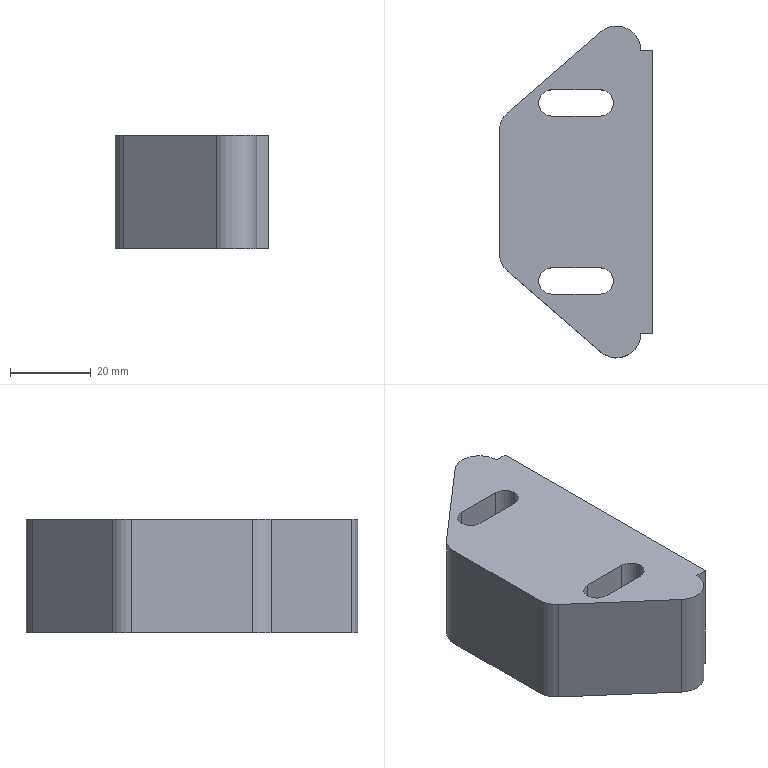Component | SolidWorks | SynchronousBeltPressingBlock-1 | 1 solid | 21 faces | box 37.99 x 82 x 28 mm | volume 62042 mm3 | plane 12 | cylinder 9 | commonest cylinder face diameters 12 x5 6.5 x4
build123d program:
from build123d import *

# Parameters (mm, degrees)
BOSS_EXTRUDE1_DEPTH              = 28
SKETCH1_W                        = 70
SKETCH1_H                        = 3.49
PRESSING_SURFACE_EXTENSION_DEPTH = 14


with BuildPart() as part:
    # Sketch1_2 → Boss-Extrude1 (new body)
    with BuildSketch(Plane(origin=(0, 0, -14), x_dir=(-1, 0, 0), z_dir=(0, 0, -1))):
        with BuildLine():
            Line((35, 0), (-35, 0))
            ThreePointArc((-35, 0), (-40.46, -3.512), (-39.528, -9.937))
            Line((-39.528, -9.937), (-19.528, -32.937))
            ThreePointArc((-19.528, -32.937), (-17.488, -34.46), (-15, -35))
            Line((-15, -35), (15, -35))
            ThreePointArc((15, -35), (17.488, -34.46), (19.528, -32.937))
            Line((19.528, -32.937), (39.528, -9.937))
            ThreePointArc((39.528, -9.937), (40.46, -3.512), (35, 0))
        make_face()
        with BuildLine():
            Line((18.75, -22), (18.75, -10))
            ThreePointArc((18.75, -10), (22, -6.75), (25.25, -10))
            Line((25.25, -10), (25.25, -22))
            ThreePointArc((25.25, -22), (22, -25.25), (18.75, -22))
        make_face(mode=Mode.SUBTRACT)
        with BuildLine():
            Line((-25.25, -22), (-25.25, -10))
            ThreePointArc((-25.25, -10), (-22, -6.75), (-18.75, -10))
            Line((-18.75, -10), (-18.75, -22))
            ThreePointArc((-18.75, -22), (-22, -25.25), (-25.25, -22))
        make_face(mode=Mode.SUBTRACT)
    extrude(amount=-BOSS_EXTRUDE1_DEPTH)

    # Sketch1 → Pressing Surface Extension (add, symmetric)
    with BuildSketch(Plane.XY):
        with Locations((0, 1.245)):
            Rectangle(SKETCH1_W, SKETCH1_H)
    extrude(amount=PRESSING_SURFACE_EXTENSION_DEPTH, both=True)


solid = part.part

# Placed as in the assembly
solid = solid.moved(Location((-60.431, 269, 134), (0, 0, -90)))
STEP:
#1=COLOUR_RGB('',0.7922,0.8196,0.9333);
#2=FILL_AREA_STYLE_COLOUR('',#1);
#3=FILL_AREA_STYLE('',(#2));
#4=SURFACE_STYLE_FILL_AREA(#3);
#5=SURFACE_SIDE_STYLE('',(#4));
#6=SURFACE_STYLE_USAGE(.BOTH.,#5);
#7=PRESENTATION_STYLE_ASSIGNMENT((#6));
#8=CARTESIAN_POINT('',(-2.77,12.147,5.827));
#9=VERTEX_POINT('',#8);
#10=CARTESIAN_POINT('',(-2.615,12.205,5.827));
#11=VERTEX_POINT('',#10);
#12=CARTESIAN_POINT('',(-2.615,11.969,5.827));
#13=DIRECTION('',(0.,0.,-1.));
#14=DIRECTION('',(0.,1.,0.));
#15=AXIS2_PLACEMENT_3D('',#12,#13,#14);
#16=CIRCLE('',#15,0.2362);
#17=EDGE_CURVE('',#9,#11,#16,.T.);
#18=ORIENTED_EDGE('',*,*,#17,.T.);
#19=CARTESIAN_POINT('',(-2.615,12.205,4.724));
#20=VERTEX_POINT('',#19);
#21=CARTESIAN_POINT('',(-2.615,12.205,5.827));
#22=DIRECTION('',(0.,0.,-1.));
#23=VECTOR('',#22,39.37);
#24=LINE('',#21,#23);
#25=EDGE_CURVE('',#11,#20,#24,.T.);
#26=ORIENTED_EDGE('',*,*,#25,.T.);
#27=CARTESIAN_POINT('',(-2.77,12.147,4.724));
#28=VERTEX_POINT('',#27);
#29=CARTESIAN_POINT('',(-2.615,11.969,4.724));
#30=DIRECTION('',(0.,0.,-1.));
#31=DIRECTION('',(0.,1.,0.));
#32=AXIS2_PLACEMENT_3D('',#29,#30,#31);
#33=CIRCLE('',#32,0.2362);
#34=EDGE_CURVE('',#28,#20,#33,.T.);
#35=ORIENTED_EDGE('',*,*,#34,.F.);
#36=CARTESIAN_POINT('',(-2.77,12.147,5.827));
#37=DIRECTION('',(0.,0.,-1.));
#38=VECTOR('',#37,39.37);
#39=LINE('',#36,#38);
#40=EDGE_CURVE('',#9,#28,#39,.T.);
#41=ORIENTED_EDGE('',*,*,#40,.F.);
#42=EDGE_LOOP('',(#18,#26,#35,#41));
#43=FACE_OUTER_BOUND('',#42,.T.);
#44=CARTESIAN_POINT('',(-2.615,11.969,5.827));
#45=DIRECTION('',(0.,0.,-1.));
#46=DIRECTION('',(0.,1.,0.));
#47=AXIS2_PLACEMENT_3D('',#44,#45,#46);
#48=CYLINDRICAL_SURFACE('',#47,0.2362);
#49=ADVANCED_FACE('',(#43),#48,.T.);
#50=ORIENTED_EDGE('',*,*,#25,.F.);
#51=CARTESIAN_POINT('',(-2.379,11.969,5.827));
#52=VERTEX_POINT('',#51);
#53=CARTESIAN_POINT('',(-2.615,11.969,5.827));
#54=DIRECTION('',(0.,0.,-1.));
#55=DIRECTION('',(0.,1.,0.));
#56=AXIS2_PLACEMENT_3D('',#53,#54,#55);
#57=CIRCLE('',#56,0.2362);
#58=EDGE_CURVE('',#11,#52,#57,.T.);
#59=ORIENTED_EDGE('',*,*,#58,.T.);
#60=CARTESIAN_POINT('',(-2.379,11.969,4.724));
#61=VERTEX_POINT('',#60);
#62=CARTESIAN_POINT('',(-2.379,11.969,5.827));
#63=DIRECTION('',(0.,0.,-1.));
#64=VECTOR('',#63,39.37);
#65=LINE('',#62,#64);
#66=EDGE_CURVE('',#52,#61,#65,.T.);
#67=ORIENTED_EDGE('',*,*,#66,.T.);
#68=CARTESIAN_POINT('',(-2.615,11.969,4.724));
#69=DIRECTION('',(0.,0.,-1.));
#70=DIRECTION('',(0.,1.,0.));
#71=AXIS2_PLACEMENT_3D('',#68,#69,#70);
#72=CIRCLE('',#71,0.2362);
#73=EDGE_CURVE('',#20,#61,#72,.T.);
#74=ORIENTED_EDGE('',*,*,#73,.F.);
#75=EDGE_LOOP('',(#50,#59,#67,#74));
#76=FACE_OUTER_BOUND('',#75,.T.);
#77=CARTESIAN_POINT('',(-2.615,11.969,5.827));
#78=DIRECTION('',(0.,0.,-1.));
#79=DIRECTION('',(0.,1.,0.));
#80=AXIS2_PLACEMENT_3D('',#77,#78,#79);
#81=CYLINDRICAL_SURFACE('',#80,0.2362);
#82=ADVANCED_FACE('',(#76),#81,.T.);
#83=CARTESIAN_POINT('',(-3.676,11.359,4.724));
#84=VERTEX_POINT('',#83);
#85=CARTESIAN_POINT('',(-3.676,11.359,4.724));
#86=DIRECTION('',(0.7546,0.6562,0.));
#87=VECTOR('',#86,39.37);
#88=LINE('',#85,#87);
#89=EDGE_CURVE('',#84,#28,#88,.T.);
#90=ORIENTED_EDGE('',*,*,#89,.F.);
#91=CARTESIAN_POINT('',(-3.676,11.359,5.827));
#92=VERTEX_POINT('',#91);
#93=CARTESIAN_POINT('',(-3.676,11.359,5.827));
#94=DIRECTION('',(0.,0.,-1.));
#95=VECTOR('',#94,39.37);
#96=LINE('',#93,#95);
#97=EDGE_CURVE('',#92,#84,#96,.T.);
#98=ORIENTED_EDGE('',*,*,#97,.F.);
#99=CARTESIAN_POINT('',(-3.676,11.359,5.827));
#100=DIRECTION('',(0.7546,0.6562,0.));
#101=VECTOR('',#100,39.37);
#102=LINE('',#99,#101);
#103=EDGE_CURVE('',#92,#9,#102,.T.);
#104=ORIENTED_EDGE('',*,*,#103,.T.);
#105=ORIENTED_EDGE('',*,*,#40,.T.);
#106=EDGE_LOOP('',(#90,#98,#104,#105));
#107=FACE_OUTER_BOUND('',#106,.T.);
#108=CARTESIAN_POINT('',(-3.676,11.359,5.827));
#109=DIRECTION('',(-0.6562,0.7546,0.));
#110=DIRECTION('',(-0.7546,-0.6562,0.));
#111=AXIS2_PLACEMENT_3D('',#108,#109,#110);
#112=PLANE('',#111);
#113=ADVANCED_FACE('',(#107),#112,.T.);
#114=CARTESIAN_POINT('',(-3.757,11.181,4.724));
#115=VERTEX_POINT('',#114);
#116=CARTESIAN_POINT('',(-3.521,11.181,4.724));
#117=DIRECTION('',(0.,0.,-1.));
#118=DIRECTION('',(0.,1.,0.));
#119=AXIS2_PLACEMENT_3D('',#116,#117,#118);
#120=CIRCLE('',#119,0.2362);
#121=EDGE_CURVE('',#115,#84,#120,.T.);
#122=ORIENTED_EDGE('',*,*,#121,.F.);
#123=CARTESIAN_POINT('',(-3.757,11.181,5.827));
#124=VERTEX_POINT('',#123);
#125=CARTESIAN_POINT('',(-3.757,11.181,5.827));
#126=DIRECTION('',(0.,0.,-1.));
#127=VECTOR('',#126,39.37);
#128=LINE('',#125,#127);
#129=EDGE_CURVE('',#124,#115,#128,.T.);
#130=ORIENTED_EDGE('',*,*,#129,.F.);
#131=CARTESIAN_POINT('',(-3.521,11.181,5.827));
#132=DIRECTION('',(0.,0.,-1.));
#133=DIRECTION('',(0.,1.,0.));
#134=AXIS2_PLACEMENT_3D('',#131,#132,#133);
#135=CIRCLE('',#134,0.2362);
#136=EDGE_CURVE('',#124,#92,#135,.T.);
#137=ORIENTED_EDGE('',*,*,#136,.T.);
#138=ORIENTED_EDGE('',*,*,#97,.T.);
#139=EDGE_LOOP('',(#122,#130,#137,#138));
#140=FACE_OUTER_BOUND('',#139,.T.);
#141=CARTESIAN_POINT('',(-3.521,11.181,5.827));
#142=DIRECTION('',(0.,0.,-1.));
#143=DIRECTION('',(0.,1.,0.));
#144=AXIS2_PLACEMENT_3D('',#141,#142,#143);
#145=CYLINDRICAL_SURFACE('',#144,0.2362);
#146=ADVANCED_FACE('',(#140),#145,.T.);
#147=CARTESIAN_POINT('',(-3.757,10.,4.724));
#148=VERTEX_POINT('',#147);
#149=CARTESIAN_POINT('',(-3.757,10.,4.724));
#150=DIRECTION('',(0.,1.,0.));
#151=VECTOR('',#150,39.37);
#152=LINE('',#149,#151);
#153=EDGE_CURVE('',#148,#115,#152,.T.);
#154=ORIENTED_EDGE('',*,*,#153,.F.);
#155=CARTESIAN_POINT('',(-3.757,10.,5.827));
#156=VERTEX_POINT('',#155);
#157=CARTESIAN_POINT('',(-3.757,10.,5.827));
#158=DIRECTION('',(0.,0.,-1.));
#159=VECTOR('',#158,39.37);
#160=LINE('',#157,#159);
#161=EDGE_CURVE('',#156,#148,#160,.T.);
#162=ORIENTED_EDGE('',*,*,#161,.F.);
#163=CARTESIAN_POINT('',(-3.757,10.,5.827));
#164=DIRECTION('',(0.,1.,0.));
#165=VECTOR('',#164,39.37);
#166=LINE('',#163,#165);
#167=EDGE_CURVE('',#156,#124,#166,.T.);
#168=ORIENTED_EDGE('',*,*,#167,.T.);
#169=ORIENTED_EDGE('',*,*,#129,.T.);
#170=EDGE_LOOP('',(#154,#162,#168,#169));
#171=FACE_OUTER_BOUND('',#170,.T.);
#172=CARTESIAN_POINT('',(-3.757,10.,5.827));
#173=DIRECTION('',(-1.,0.,0.));
#174=DIRECTION('',(0.,0.,-1.));
#175=AXIS2_PLACEMENT_3D('',#172,#173,#174);
#176=PLANE('',#175);
#177=ADVANCED_FACE('',(#171),#176,.T.);
#178=CARTESIAN_POINT('',(-3.676,9.822,4.724));
#179=VERTEX_POINT('',#178);
#180=CARTESIAN_POINT('',(-3.521,10.,4.724));
#181=DIRECTION('',(0.,0.,-1.));
#182=DIRECTION('',(0.,1.,0.));
#183=AXIS2_PLACEMENT_3D('',#180,#181,#182);
#184=CIRCLE('',#183,0.2362);
#185=EDGE_CURVE('',#179,#148,#184,.T.);
#186=ORIENTED_EDGE('',*,*,#185,.F.);
#187=CARTESIAN_POINT('',(-3.676,9.822,5.827));
#188=VERTEX_POINT('',#187);
#189=CARTESIAN_POINT('',(-3.676,9.822,5.827));
#190=DIRECTION('',(0.,0.,-1.));
#191=VECTOR('',#190,39.37);
#192=LINE('',#189,#191);
#193=EDGE_CURVE('',#188,#179,#192,.T.);
#194=ORIENTED_EDGE('',*,*,#193,.F.);
#195=CARTESIAN_POINT('',(-3.521,10.,5.827));
#196=DIRECTION('',(0.,0.,-1.));
#197=DIRECTION('',(0.,1.,0.));
#198=AXIS2_PLACEMENT_3D('',#195,#196,#197);
#199=CIRCLE('',#198,0.2362);
#200=EDGE_CURVE('',#188,#156,#199,.T.);
#201=ORIENTED_EDGE('',*,*,#200,.T.);
#202=ORIENTED_EDGE('',*,*,#161,.T.);
#203=EDGE_LOOP('',(#186,#194,#201,#202));
#204=FACE_OUTER_BOUND('',#203,.T.);
#205=CARTESIAN_POINT('',(-3.521,10.,5.827));
#206=DIRECTION('',(0.,0.,-1.));
#207=DIRECTION('',(0.,1.,0.));
#208=AXIS2_PLACEMENT_3D('',#205,#206,#207);
#209=CYLINDRICAL_SURFACE('',#208,0.2362);
#210=ADVANCED_FACE('',(#204),#209,.T.);
#211=CARTESIAN_POINT('',(-2.77,9.034,4.724));
#212=VERTEX_POINT('',#211);
#213=CARTESIAN_POINT('',(-2.77,9.034,4.724));
#214=DIRECTION('',(-0.7546,0.6562,0.));
#215=VECTOR('',#214,39.37);
#216=LINE('',#213,#215);
#217=EDGE_CURVE('',#212,#179,#216,.T.);
#218=ORIENTED_EDGE('',*,*,#217,.F.);
#219=CARTESIAN_POINT('',(-2.77,9.034,5.827));
#220=VERTEX_POINT('',#219);
#221=CARTESIAN_POINT('',(-2.77,9.034,5.827));
#222=DIRECTION('',(0.,0.,-1.));
#223=VECTOR('',#222,39.37);
#224=LINE('',#221,#223);
#225=EDGE_CURVE('',#220,#212,#224,.T.);
#226=ORIENTED_EDGE('',*,*,#225,.F.);
#227=CARTESIAN_POINT('',(-2.77,9.034,5.827));
#228=DIRECTION('',(-0.7546,0.6562,0.));
#229=VECTOR('',#228,39.37);
#230=LINE('',#227,#229);
#231=EDGE_CURVE('',#220,#188,#230,.T.);
#232=ORIENTED_EDGE('',*,*,#231,.T.);
#233=ORIENTED_EDGE('',*,*,#193,.T.);
#234=EDGE_LOOP('',(#218,#226,#232,#233));
#235=FACE_OUTER_BOUND('',#234,.T.);
#236=CARTESIAN_POINT('',(-2.77,9.034,5.827));
#237=DIRECTION('',(-0.6562,-0.7546,0.));
#238=DIRECTION('',(0.7546,-0.6562,0.));
#239=AXIS2_PLACEMENT_3D('',#236,#237,#238);
#240=PLANE('',#239);
#241=ADVANCED_FACE('',(#235),#240,.T.);
#242=CARTESIAN_POINT('',(-2.379,9.213,4.724));
#243=VERTEX_POINT('',#242);
#244=CARTESIAN_POINT('',(-2.615,9.213,4.724));
#245=DIRECTION('',(0.,0.,-1.));
#246=DIRECTION('',(0.,1.,0.));
#247=AXIS2_PLACEMENT_3D('',#244,#245,#246);
#248=CIRCLE('',#247,0.2362);
#249=EDGE_CURVE('',#243,#212,#248,.T.);
#250=ORIENTED_EDGE('',*,*,#249,.F.);
#251=CARTESIAN_POINT('',(-2.379,9.213,5.827));
#252=VERTEX_POINT('',#251);
#253=CARTESIAN_POINT('',(-2.379,9.213,5.827));
#254=DIRECTION('',(0.,0.,-1.));
#255=VECTOR('',#254,39.37);
#256=LINE('',#253,#255);
#257=EDGE_CURVE('',#252,#243,#256,.T.);
#258=ORIENTED_EDGE('',*,*,#257,.F.);
#259=CARTESIAN_POINT('',(-2.615,9.213,5.827));
#260=DIRECTION('',(0.,0.,-1.));
#261=DIRECTION('',(0.,1.,0.));
#262=AXIS2_PLACEMENT_3D('',#259,#260,#261);
#263=CIRCLE('',#262,0.2362);
#264=EDGE_CURVE('',#252,#220,#263,.T.);
#265=ORIENTED_EDGE('',*,*,#264,.T.);
#266=ORIENTED_EDGE('',*,*,#225,.T.);
#267=EDGE_LOOP('',(#250,#258,#265,#266));
#268=FACE_OUTER_BOUND('',#267,.T.);
#269=CARTESIAN_POINT('',(-2.615,9.213,5.827));
#270=DIRECTION('',(0.,0.,-1.));
#271=DIRECTION('',(0.,1.,0.));
#272=AXIS2_PLACEMENT_3D('',#269,#270,#271);
#273=CYLINDRICAL_SURFACE('',#272,0.2362);
#274=ADVANCED_FACE('',(#268),#273,.T.);
#275=ORIENTED_EDGE('',*,*,#264,.F.);
#276=CARTESIAN_POINT('',(-2.261,9.213,5.827));
#277=VERTEX_POINT('',#276);
#278=CARTESIAN_POINT('',(-2.399,9.213,5.827));
#279=DIRECTION('',(1.,-0.,0.));
#280=VECTOR('',#279,39.37);
#281=LINE('',#278,#280);
#282=EDGE_CURVE('',#252,#277,#281,.T.);
#283=ORIENTED_EDGE('',*,*,#282,.T.);
#284=CARTESIAN_POINT('',(-2.261,11.969,5.827));
#285=VERTEX_POINT('',#284);
#286=CARTESIAN_POINT('',(-2.261,9.213,5.827));
#287=DIRECTION('',(0.,1.,0.));
#288=VECTOR('',#287,39.37);
#289=LINE('',#286,#288);
#290=EDGE_CURVE('',#277,#285,#289,.T.);
#291=ORIENTED_EDGE('',*,*,#290,.T.);
#292=CARTESIAN_POINT('',(-2.261,11.969,5.827));
#293=DIRECTION('',(-1.,0.,0.));
#294=VECTOR('',#293,39.37);
#295=LINE('',#292,#294);
#296=EDGE_CURVE('',#285,#52,#295,.T.);
#297=ORIENTED_EDGE('',*,*,#296,.T.);
#298=ORIENTED_EDGE('',*,*,#58,.F.);
#299=ORIENTED_EDGE('',*,*,#17,.F.);
#300=ORIENTED_EDGE('',*,*,#103,.F.);
#301=ORIENTED_EDGE('',*,*,#136,.F.);
#302=ORIENTED_EDGE('',*,*,#167,.F.);
#303=ORIENTED_EDGE('',*,*,#200,.F.);
#304=ORIENTED_EDGE('',*,*,#231,.F.);
#305=EDGE_LOOP('',(#275,#283,#291,#297,#298,#299,#300,#301,#302,#303,#304));
#306=FACE_OUTER_BOUND('',#305,.T.);
#307=CARTESIAN_POINT('',(-2.773,11.329,5.827));
#308=VERTEX_POINT('',#307);
#309=CARTESIAN_POINT('',(-3.245,11.329,5.827));
#310=VERTEX_POINT('',#309);
#311=CARTESIAN_POINT('',(-3.245,11.329,5.827));
#312=DIRECTION('',(-1.,0.,0.));
#313=VECTOR('',#312,39.37);
#314=LINE('',#311,#313);
#315=EDGE_CURVE('',#308,#310,#314,.T.);
#316=ORIENTED_EDGE('',*,*,#315,.T.);
#317=CARTESIAN_POINT('',(-3.245,11.585,5.827));
#318=VERTEX_POINT('',#317);
#319=CARTESIAN_POINT('',(-3.245,11.457,5.827));
#320=DIRECTION('',(0.,0.,-1.));
#321=DIRECTION('',(0.,-1.,0.));
#322=AXIS2_PLACEMENT_3D('',#319,#320,#321);
#323=CIRCLE('',#322,0.128);
#324=EDGE_CURVE('',#310,#318,#323,.T.);
#325=ORIENTED_EDGE('',*,*,#324,.T.);
#326=CARTESIAN_POINT('',(-2.773,11.585,5.827));
#327=VERTEX_POINT('',#326);
#328=CARTESIAN_POINT('',(-2.773,11.585,5.827));
#329=DIRECTION('',(1.,-0.,0.));
#330=VECTOR('',#329,39.37);
#331=LINE('',#328,#330);
#332=EDGE_CURVE('',#318,#327,#331,.T.);
#333=ORIENTED_EDGE('',*,*,#332,.T.);
#334=CARTESIAN_POINT('',(-2.773,11.457,5.827));
#335=DIRECTION('',(0.,0.,-1.));
#336=DIRECTION('',(0.,-1.,0.));
#337=AXIS2_PLACEMENT_3D('',#334,#335,#336);
#338=CIRCLE('',#337,0.128);
#339=EDGE_CURVE('',#327,#308,#338,.T.);
#340=ORIENTED_EDGE('',*,*,#339,.T.);
#341=EDGE_LOOP('',(#316,#325,#333,#340));
#342=FACE_BOUND('',#341,.T.);
#343=CARTESIAN_POINT('',(-2.773,9.596,5.827));
#344=VERTEX_POINT('',#343);
#345=CARTESIAN_POINT('',(-3.245,9.596,5.827));
#346=VERTEX_POINT('',#345);
#347=CARTESIAN_POINT('',(-3.245,9.596,5.827));
#348=DIRECTION('',(-1.,0.,0.));
#349=VECTOR('',#348,39.37);
#350=LINE('',#347,#349);
#351=EDGE_CURVE('',#344,#346,#350,.T.);
#352=ORIENTED_EDGE('',*,*,#351,.T.);
#353=CARTESIAN_POINT('',(-3.245,9.852,5.827));
#354=VERTEX_POINT('',#353);
#355=CARTESIAN_POINT('',(-3.245,9.724,5.827));
#356=DIRECTION('',(0.,0.,-1.));
#357=DIRECTION('',(0.,-1.,0.));
#358=AXIS2_PLACEMENT_3D('',#355,#356,#357);
#359=CIRCLE('',#358,0.128);
#360=EDGE_CURVE('',#346,#354,#359,.T.);
#361=ORIENTED_EDGE('',*,*,#360,.T.);
#362=CARTESIAN_POINT('',(-2.773,9.852,5.827));
#363=VERTEX_POINT('',#362);
#364=CARTESIAN_POINT('',(-2.773,9.852,5.827));
#365=DIRECTION('',(1.,-0.,0.));
#366=VECTOR('',#365,39.37);
#367=LINE('',#364,#366);
#368=EDGE_CURVE('',#354,#363,#367,.T.);
#369=ORIENTED_EDGE('',*,*,#368,.T.);
#370=CARTESIAN_POINT('',(-2.773,9.724,5.827));
#371=DIRECTION('',(0.,0.,-1.));
#372=DIRECTION('',(0.,-1.,0.));
#373=AXIS2_PLACEMENT_3D('',#370,#371,#372);
#374=CIRCLE('',#373,0.128);
#375=EDGE_CURVE('',#363,#344,#374,.T.);
#376=ORIENTED_EDGE('',*,*,#375,.T.);
#377=EDGE_LOOP('',(#352,#361,#369,#376));
#378=FACE_BOUND('',#377,.T.);
#379=CARTESIAN_POINT('',(-2.615,11.969,5.827));
#380=DIRECTION('',(0.,0.,-1.));
#381=DIRECTION('',(0.,1.,0.));
#382=AXIS2_PLACEMENT_3D('',#379,#380,#381);
#383=PLANE('',#382);
#384=ADVANCED_FACE('',(#306,#342,#378),#383,.F.);
#385=ORIENTED_EDGE('',*,*,#34,.T.);
#386=ORIENTED_EDGE('',*,*,#73,.T.);
#387=CARTESIAN_POINT('',(-2.261,11.969,4.724));
#388=VERTEX_POINT('',#387);
#389=CARTESIAN_POINT('',(-2.261,11.969,4.724));
#390=DIRECTION('',(-1.,0.,0.));
#391=VECTOR('',#390,39.37);
#392=LINE('',#389,#391);
#393=EDGE_CURVE('',#388,#61,#392,.T.);
#394=ORIENTED_EDGE('',*,*,#393,.F.);
#395=CARTESIAN_POINT('',(-2.261,9.213,4.724));
#396=VERTEX_POINT('',#395);
#397=CARTESIAN_POINT('',(-2.261,9.213,4.724));
#398=DIRECTION('',(0.,1.,0.));
#399=VECTOR('',#398,39.37);
#400=LINE('',#397,#399);
#401=EDGE_CURVE('',#396,#388,#400,.T.);
#402=ORIENTED_EDGE('',*,*,#401,.F.);
#403=CARTESIAN_POINT('',(-2.399,9.213,4.724));
#404=DIRECTION('',(1.,-0.,0.));
#405=VECTOR('',#404,39.37);
#406=LINE('',#403,#405);
#407=EDGE_CURVE('',#243,#396,#406,.T.);
#408=ORIENTED_EDGE('',*,*,#407,.F.);
#409=ORIENTED_EDGE('',*,*,#249,.T.);
#410=ORIENTED_EDGE('',*,*,#217,.T.);
#411=ORIENTED_EDGE('',*,*,#185,.T.);
#412=ORIENTED_EDGE('',*,*,#153,.T.);
#413=ORIENTED_EDGE('',*,*,#121,.T.);
#414=ORIENTED_EDGE('',*,*,#89,.T.);
#415=EDGE_LOOP('',(#385,#386,#394,#402,#408,#409,#410,#411,#412,#413,#414));
#416=FACE_OUTER_BOUND('',#415,.T.);
#417=CARTESIAN_POINT('',(-3.245,9.596,4.724));
#418=VERTEX_POINT('',#417);
#419=CARTESIAN_POINT('',(-3.245,9.852,4.724));
#420=VERTEX_POINT('',#419);
#421=CARTESIAN_POINT('',(-3.245,9.724,4.724));
#422=DIRECTION('',(0.,0.,-1.));
#423=DIRECTION('',(0.,-1.,0.));
#424=AXIS2_PLACEMENT_3D('',#421,#422,#423);
#425=CIRCLE('',#424,0.128);
#426=EDGE_CURVE('',#418,#420,#425,.T.);
#427=ORIENTED_EDGE('',*,*,#426,.F.);
#428=CARTESIAN_POINT('',(-2.773,9.596,4.724));
#429=VERTEX_POINT('',#428);
#430=CARTESIAN_POINT('',(-3.245,9.596,4.724));
#431=DIRECTION('',(-1.,0.,0.));
#432=VECTOR('',#431,39.37);
#433=LINE('',#430,#432);
#434=EDGE_CURVE('',#429,#418,#433,.T.);
#435=ORIENTED_EDGE('',*,*,#434,.F.);
#436=CARTESIAN_POINT('',(-2.773,9.852,4.724));
#437=VERTEX_POINT('',#436);
#438=CARTESIAN_POINT('',(-2.773,9.724,4.724));
#439=DIRECTION('',(0.,0.,-1.));
#440=DIRECTION('',(0.,-1.,0.));
#441=AXIS2_PLACEMENT_3D('',#438,#439,#440);
#442=CIRCLE('',#441,0.128);
#443=EDGE_CURVE('',#437,#429,#442,.T.);
#444=ORIENTED_EDGE('',*,*,#443,.F.);
#445=CARTESIAN_POINT('',(-2.773,9.852,4.724));
#446=DIRECTION('',(1.,-0.,0.));
#447=VECTOR('',#446,39.37);
#448=LINE('',#445,#447);
#449=EDGE_CURVE('',#420,#437,#448,.T.);
#450=ORIENTED_EDGE('',*,*,#449,.F.);
#451=EDGE_LOOP('',(#427,#435,#444,#450));
#452=FACE_BOUND('',#451,.T.);
#453=CARTESIAN_POINT('',(-3.245,11.329,4.724));
#454=VERTEX_POINT('',#453);
#455=CARTESIAN_POINT('',(-3.245,11.585,4.724));
#456=VERTEX_POINT('',#455);
#457=CARTESIAN_POINT('',(-3.245,11.457,4.724));
#458=DIRECTION('',(0.,0.,-1.));
#459=DIRECTION('',(0.,-1.,0.));
#460=AXIS2_PLACEMENT_3D('',#457,#458,#459);
#461=CIRCLE('',#460,0.128);
#462=EDGE_CURVE('',#454,#456,#461,.T.);
#463=ORIENTED_EDGE('',*,*,#462,.F.);
#464=CARTESIAN_POINT('',(-2.773,11.329,4.724));
#465=VERTEX_POINT('',#464);
#466=CARTESIAN_POINT('',(-3.245,11.329,4.724));
#467=DIRECTION('',(-1.,0.,0.));
#468=VECTOR('',#467,39.37);
#469=LINE('',#466,#468);
#470=EDGE_CURVE('',#465,#454,#469,.T.);
#471=ORIENTED_EDGE('',*,*,#470,.F.);
#472=CARTESIAN_POINT('',(-2.773,11.585,4.724));
#473=VERTEX_POINT('',#472);
#474=CARTESIAN_POINT('',(-2.773,11.457,4.724));
#475=DIRECTION('',(0.,0.,-1.));
#476=DIRECTION('',(0.,-1.,0.));
#477=AXIS2_PLACEMENT_3D('',#474,#475,#476);
#478=CIRCLE('',#477,0.128);
#479=EDGE_CURVE('',#473,#465,#478,.T.);
#480=ORIENTED_EDGE('',*,*,#479,.F.);
#481=CARTESIAN_POINT('',(-2.773,11.585,4.724));
#482=DIRECTION('',(1.,-0.,0.));
#483=VECTOR('',#482,39.37);
#484=LINE('',#481,#483);
#485=EDGE_CURVE('',#456,#473,#484,.T.);
#486=ORIENTED_EDGE('',*,*,#485,.F.);
#487=EDGE_LOOP('',(#463,#471,#480,#486));
#488=FACE_BOUND('',#487,.T.);
#489=CARTESIAN_POINT('',(-2.615,11.969,4.724));
#490=DIRECTION('',(0.,0.,-1.));
#491=DIRECTION('',(0.,1.,0.));
#492=AXIS2_PLACEMENT_3D('',#489,#490,#491);
#493=PLANE('',#492);
#494=ADVANCED_FACE('',(#416,#452,#488),#493,.T.);
#495=ORIENTED_EDGE('',*,*,#462,.T.);
#496=CARTESIAN_POINT('',(-3.245,11.585,5.827));
#497=DIRECTION('',(0.,0.,-1.));
#498=VECTOR('',#497,39.37);
#499=LINE('',#496,#498);
#500=EDGE_CURVE('',#318,#456,#499,.T.);
#501=ORIENTED_EDGE('',*,*,#500,.F.);
#502=ORIENTED_EDGE('',*,*,#324,.F.);
#503=CARTESIAN_POINT('',(-3.245,11.329,5.827));
#504=DIRECTION('',(0.,0.,-1.));
#505=VECTOR('',#504,39.37);
#506=LINE('',#503,#505);
#507=EDGE_CURVE('',#310,#454,#506,.T.);
#508=ORIENTED_EDGE('',*,*,#507,.T.);
#509=EDGE_LOOP('',(#495,#501,#502,#508));
#510=FACE_OUTER_BOUND('',#509,.T.);
#511=CARTESIAN_POINT('',(-3.245,11.457,5.827));
#512=DIRECTION('',(0.,0.,-1.));
#513=DIRECTION('',(0.,1.,0.));
#514=AXIS2_PLACEMENT_3D('',#511,#512,#513);
#515=CYLINDRICAL_SURFACE('',#514,0.128);
#516=ADVANCED_FACE('',(#510),#515,.F.);
#517=ORIENTED_EDGE('',*,*,#470,.T.);
#518=ORIENTED_EDGE('',*,*,#507,.F.);
#519=ORIENTED_EDGE('',*,*,#315,.F.);
#520=CARTESIAN_POINT('',(-2.773,11.329,5.827));
#521=DIRECTION('',(0.,0.,-1.));
#522=VECTOR('',#521,39.37);
#523=LINE('',#520,#522);
#524=EDGE_CURVE('',#308,#465,#523,.T.);
#525=ORIENTED_EDGE('',*,*,#524,.T.);
#526=EDGE_LOOP('',(#517,#518,#519,#525));
#527=FACE_OUTER_BOUND('',#526,.T.);
#528=CARTESIAN_POINT('',(-3.245,11.329,5.827));
#529=DIRECTION('',(-0.,-1.,0.));
#530=DIRECTION('',(0.,0.,-1.));
#531=AXIS2_PLACEMENT_3D('',#528,#529,#530);
#532=PLANE('',#531);
#533=ADVANCED_FACE('',(#527),#532,.F.);
#534=ORIENTED_EDGE('',*,*,#479,.T.);
#535=ORIENTED_EDGE('',*,*,#524,.F.);
#536=ORIENTED_EDGE('',*,*,#339,.F.);
#537=CARTESIAN_POINT('',(-2.773,11.585,5.827));
#538=DIRECTION('',(0.,0.,-1.));
#539=VECTOR('',#538,39.37);
#540=LINE('',#537,#539);
#541=EDGE_CURVE('',#327,#473,#540,.T.);
#542=ORIENTED_EDGE('',*,*,#541,.T.);
#543=EDGE_LOOP('',(#534,#535,#536,#542));
#544=FACE_OUTER_BOUND('',#543,.T.);
#545=CARTESIAN_POINT('',(-2.773,11.457,5.827));
#546=DIRECTION('',(0.,0.,-1.));
#547=DIRECTION('',(0.,1.,0.));
#548=AXIS2_PLACEMENT_3D('',#545,#546,#547);
#549=CYLINDRICAL_SURFACE('',#548,0.128);
#550=ADVANCED_FACE('',(#544),#549,.F.);
#551=ORIENTED_EDGE('',*,*,#485,.T.);
#552=ORIENTED_EDGE('',*,*,#541,.F.);
#553=ORIENTED_EDGE('',*,*,#332,.F.);
#554=ORIENTED_EDGE('',*,*,#500,.T.);
#555=EDGE_LOOP('',(#551,#552,#553,#554));
#556=FACE_OUTER_BOUND('',#555,.T.);
#557=CARTESIAN_POINT('',(-2.773,11.585,5.827));
#558=DIRECTION('',(0.,1.,0.));
#559=DIRECTION('',(0.,0.,1.));
#560=AXIS2_PLACEMENT_3D('',#557,#558,#559);
#561=PLANE('',#560);
#562=ADVANCED_FACE('',(#556),#561,.F.);
#563=ORIENTED_EDGE('',*,*,#426,.T.);
#564=CARTESIAN_POINT('',(-3.245,9.852,5.827));
#565=DIRECTION('',(0.,0.,-1.));
#566=VECTOR('',#565,39.37);
#567=LINE('',#564,#566);
#568=EDGE_CURVE('',#354,#420,#567,.T.);
#569=ORIENTED_EDGE('',*,*,#568,.F.);
#570=ORIENTED_EDGE('',*,*,#360,.F.);
#571=CARTESIAN_POINT('',(-3.245,9.596,5.827));
#572=DIRECTION('',(0.,0.,-1.));
#573=VECTOR('',#572,39.37);
#574=LINE('',#571,#573);
#575=EDGE_CURVE('',#346,#418,#574,.T.);
#576=ORIENTED_EDGE('',*,*,#575,.T.);
#577=EDGE_LOOP('',(#563,#569,#570,#576));
#578=FACE_OUTER_BOUND('',#577,.T.);
#579=CARTESIAN_POINT('',(-3.245,9.724,5.827));
#580=DIRECTION('',(0.,0.,-1.));
#581=DIRECTION('',(0.,1.,0.));
#582=AXIS2_PLACEMENT_3D('',#579,#580,#581);
#583=CYLINDRICAL_SURFACE('',#582,0.128);
#584=ADVANCED_FACE('',(#578),#583,.F.);
#585=ORIENTED_EDGE('',*,*,#434,.T.);
#586=ORIENTED_EDGE('',*,*,#575,.F.);
#587=ORIENTED_EDGE('',*,*,#351,.F.);
#588=CARTESIAN_POINT('',(-2.773,9.596,5.827));
#589=DIRECTION('',(0.,0.,-1.));
#590=VECTOR('',#589,39.37);
#591=LINE('',#588,#590);
#592=EDGE_CURVE('',#344,#429,#591,.T.);
#593=ORIENTED_EDGE('',*,*,#592,.T.);
#594=EDGE_LOOP('',(#585,#586,#587,#593));
#595=FACE_OUTER_BOUND('',#594,.T.);
#596=CARTESIAN_POINT('',(-3.245,9.596,5.827));
#597=DIRECTION('',(-0.,-1.,0.));
#598=DIRECTION('',(0.,0.,-1.));
#599=AXIS2_PLACEMENT_3D('',#596,#597,#598);
#600=PLANE('',#599);
#601=ADVANCED_FACE('',(#595),#600,.F.);
#602=ORIENTED_EDGE('',*,*,#443,.T.);
#603=ORIENTED_EDGE('',*,*,#592,.F.);
#604=ORIENTED_EDGE('',*,*,#375,.F.);
#605=CARTESIAN_POINT('',(-2.773,9.852,5.827));
#606=DIRECTION('',(0.,0.,-1.));
#607=VECTOR('',#606,39.37);
#608=LINE('',#605,#607);
#609=EDGE_CURVE('',#363,#437,#608,.T.);
#610=ORIENTED_EDGE('',*,*,#609,.T.);
#611=EDGE_LOOP('',(#602,#603,#604,#610));
#612=FACE_OUTER_BOUND('',#611,.T.);
#613=CARTESIAN_POINT('',(-2.773,9.724,5.827));
#614=DIRECTION('',(0.,0.,-1.));
#615=DIRECTION('',(0.,1.,0.));
#616=AXIS2_PLACEMENT_3D('',#613,#614,#615);
#617=CYLINDRICAL_SURFACE('',#616,0.128);
#618=ADVANCED_FACE('',(#612),#617,.F.);
#619=ORIENTED_EDGE('',*,*,#449,.T.);
#620=ORIENTED_EDGE('',*,*,#609,.F.);
#621=ORIENTED_EDGE('',*,*,#368,.F.);
#622=ORIENTED_EDGE('',*,*,#568,.T.);
#623=EDGE_LOOP('',(#619,#620,#621,#622));
#624=FACE_OUTER_BOUND('',#623,.T.);
#625=CARTESIAN_POINT('',(-2.773,9.852,5.827));
#626=DIRECTION('',(0.,1.,0.));
#627=DIRECTION('',(0.,0.,1.));
#628=AXIS2_PLACEMENT_3D('',#625,#626,#627);
#629=PLANE('',#628);
#630=ADVANCED_FACE('',(#624),#629,.F.);
#631=ORIENTED_EDGE('',*,*,#66,.F.);
#632=ORIENTED_EDGE('',*,*,#296,.F.);
#633=CARTESIAN_POINT('',(-2.261,11.969,5.827));
#634=DIRECTION('',(0.,0.,-1.));
#635=VECTOR('',#634,39.37);
#636=LINE('',#633,#635);
#637=EDGE_CURVE('',#285,#388,#636,.T.);
#638=ORIENTED_EDGE('',*,*,#637,.T.);
#639=ORIENTED_EDGE('',*,*,#393,.T.);
#640=EDGE_LOOP('',(#631,#632,#638,#639));
#641=FACE_OUTER_BOUND('',#640,.T.);
#642=CARTESIAN_POINT('',(-2.261,11.969,5.827));
#643=DIRECTION('',(-0.,-1.,0.));
#644=DIRECTION('',(0.,0.,-1.));
#645=AXIS2_PLACEMENT_3D('',#642,#643,#644);
#646=PLANE('',#645);
#647=ADVANCED_FACE('',(#641),#646,.F.);
#648=ORIENTED_EDGE('',*,*,#257,.T.);
#649=ORIENTED_EDGE('',*,*,#407,.T.);
#650=CARTESIAN_POINT('',(-2.261,9.213,5.827));
#651=DIRECTION('',(0.,0.,-1.));
#652=VECTOR('',#651,39.37);
#653=LINE('',#650,#652);
#654=EDGE_CURVE('',#277,#396,#653,.T.);
#655=ORIENTED_EDGE('',*,*,#654,.F.);
#656=ORIENTED_EDGE('',*,*,#282,.F.);
#657=EDGE_LOOP('',(#648,#649,#655,#656));
#658=FACE_OUTER_BOUND('',#657,.T.);
#659=CARTESIAN_POINT('',(-2.399,9.213,5.827));
#660=DIRECTION('',(0.,1.,0.));
#661=DIRECTION('',(0.,0.,1.));
#662=AXIS2_PLACEMENT_3D('',#659,#660,#661);
#663=PLANE('',#662);
#664=ADVANCED_FACE('',(#658),#663,.F.);
#665=ORIENTED_EDGE('',*,*,#401,.T.);
#666=ORIENTED_EDGE('',*,*,#637,.F.);
#667=ORIENTED_EDGE('',*,*,#290,.F.);
#668=ORIENTED_EDGE('',*,*,#654,.T.);
#669=EDGE_LOOP('',(#665,#666,#667,#668));
#670=FACE_OUTER_BOUND('',#669,.T.);
#671=CARTESIAN_POINT('',(-2.261,9.213,5.827));
#672=DIRECTION('',(-1.,0.,0.));
#673=DIRECTION('',(0.,0.,-1.));
#674=AXIS2_PLACEMENT_3D('',#671,#672,#673);
#675=PLANE('',#674);
#676=ADVANCED_FACE('',(#670),#675,.F.);
#677=CLOSED_SHELL('',(#49,#82,#113,#146,#177,#210,#241,#274,#384,#494,#516,#533,#550,#562,#584,#601,#618,#630,#647,#664,#676));
#678=MANIFOLD_SOLID_BREP('',#677);
#679=STYLED_ITEM('',(#7),#678);
#680=PRESENTATION_LAYER_ASSIGNMENT('','',(#679));
#681=CARTESIAN_POINT('',(0.,0.,0.));
#682=DIRECTION('',(0.,0.,1.));
#683=DIRECTION('',(1.,0.,0.));
#684=AXIS2_PLACEMENT_3D('',#681,#682,#683);
#685=(LENGTH_UNIT()NAMED_UNIT(*)SI_UNIT($,.METRE.));
#686=LENGTH_MEASURE_WITH_UNIT(LENGTH_MEASURE(0.0254),#685);
#687=DIMENSIONAL_EXPONENTS(1.,0.,0.,0.,0.,0.,0.);
#688=(CONVERSION_BASED_UNIT('',#686)LENGTH_UNIT()NAMED_UNIT(#687));
#689=UNCERTAINTY_MEASURE_WITH_UNIT(LENGTH_MEASURE(0.00001),#688,'','');
#690=(NAMED_UNIT(*)PLANE_ANGLE_UNIT()SI_UNIT($,.RADIAN.));
#691=(NAMED_UNIT(*)SI_UNIT($,.STERADIAN.)SOLID_ANGLE_UNIT());
#692=(GEOMETRIC_REPRESENTATION_CONTEXT(3)GLOBAL_UNCERTAINTY_ASSIGNED_CONTEXT((#689))GLOBAL_UNIT_ASSIGNED_CONTEXT((#688,#690,#691))REPRESENTATION_CONTEXT('',''));
#693=ADVANCED_BREP_SHAPE_REPRESENTATION('',(#678,#684),#692);
#694=(LENGTH_UNIT()NAMED_UNIT(*)SI_UNIT($,.METRE.));
#695=LENGTH_MEASURE_WITH_UNIT(LENGTH_MEASURE(0.0254),#694);
#696=DIMENSIONAL_EXPONENTS(1.,0.,0.,0.,0.,0.,0.);
#697=(CONVERSION_BASED_UNIT('',#695)LENGTH_UNIT()NAMED_UNIT(#696));
#698=UNCERTAINTY_MEASURE_WITH_UNIT(LENGTH_MEASURE(0.00001),#697,'','');
#699=(NAMED_UNIT(*)PLANE_ANGLE_UNIT()SI_UNIT($,.RADIAN.));
#700=(NAMED_UNIT(*)SI_UNIT($,.STERADIAN.)SOLID_ANGLE_UNIT());
#701=(GEOMETRIC_REPRESENTATION_CONTEXT(3)GLOBAL_UNCERTAINTY_ASSIGNED_CONTEXT((#698))GLOBAL_UNIT_ASSIGNED_CONTEXT((#697,#699,#700))REPRESENTATION_CONTEXT('',''));
#702=MECHANICAL_DESIGN_GEOMETRIC_PRESENTATION_REPRESENTATION('',(#679),#701);